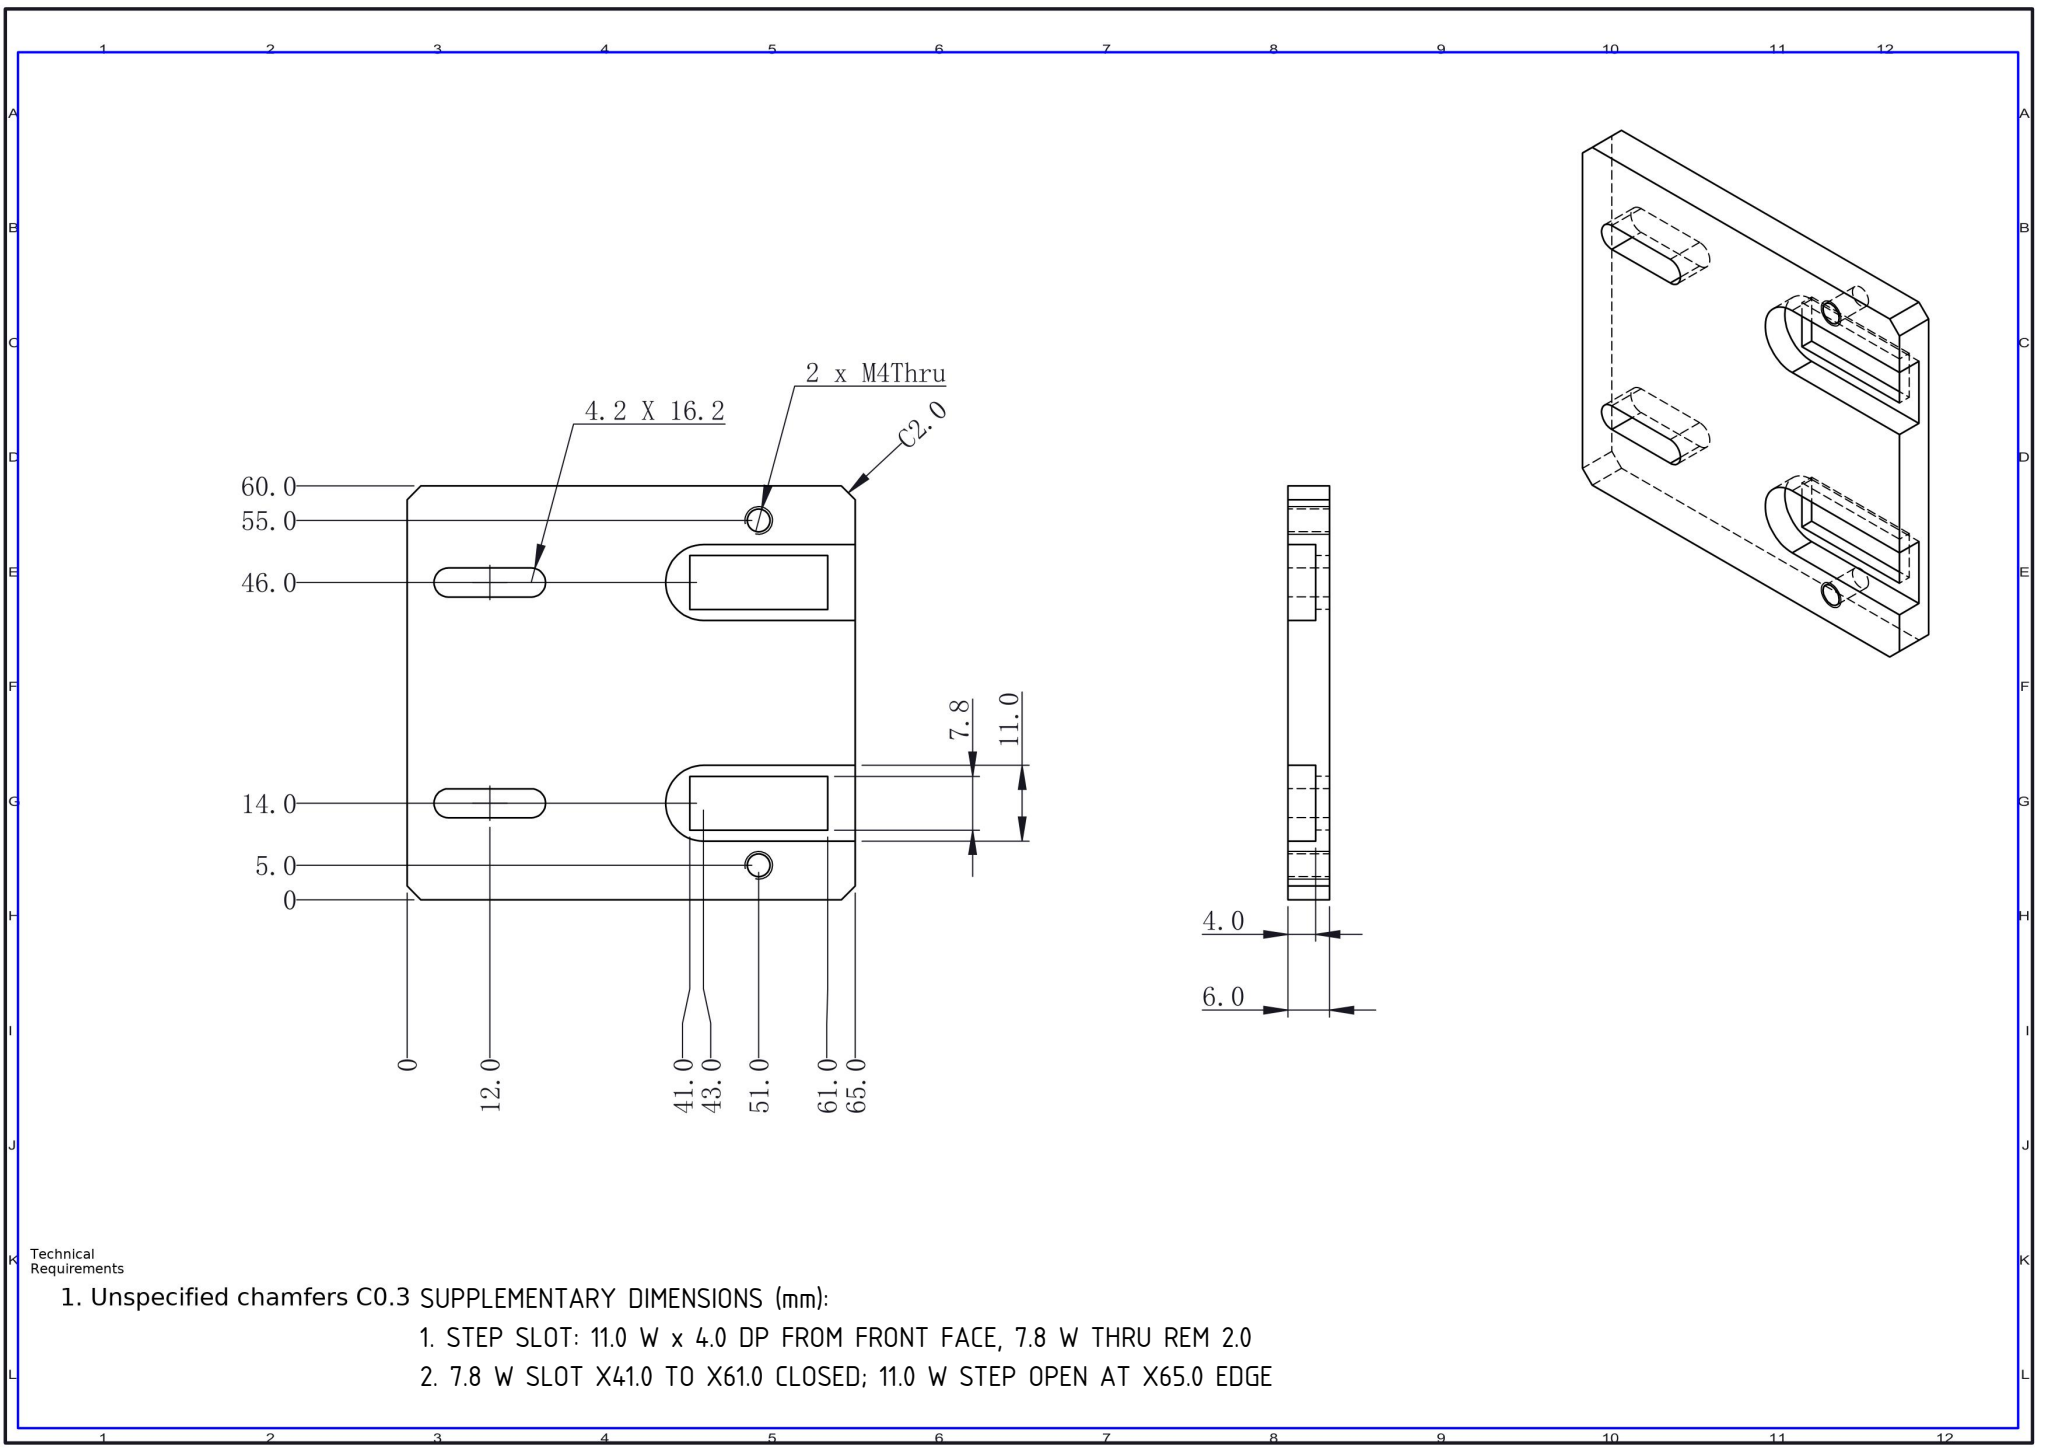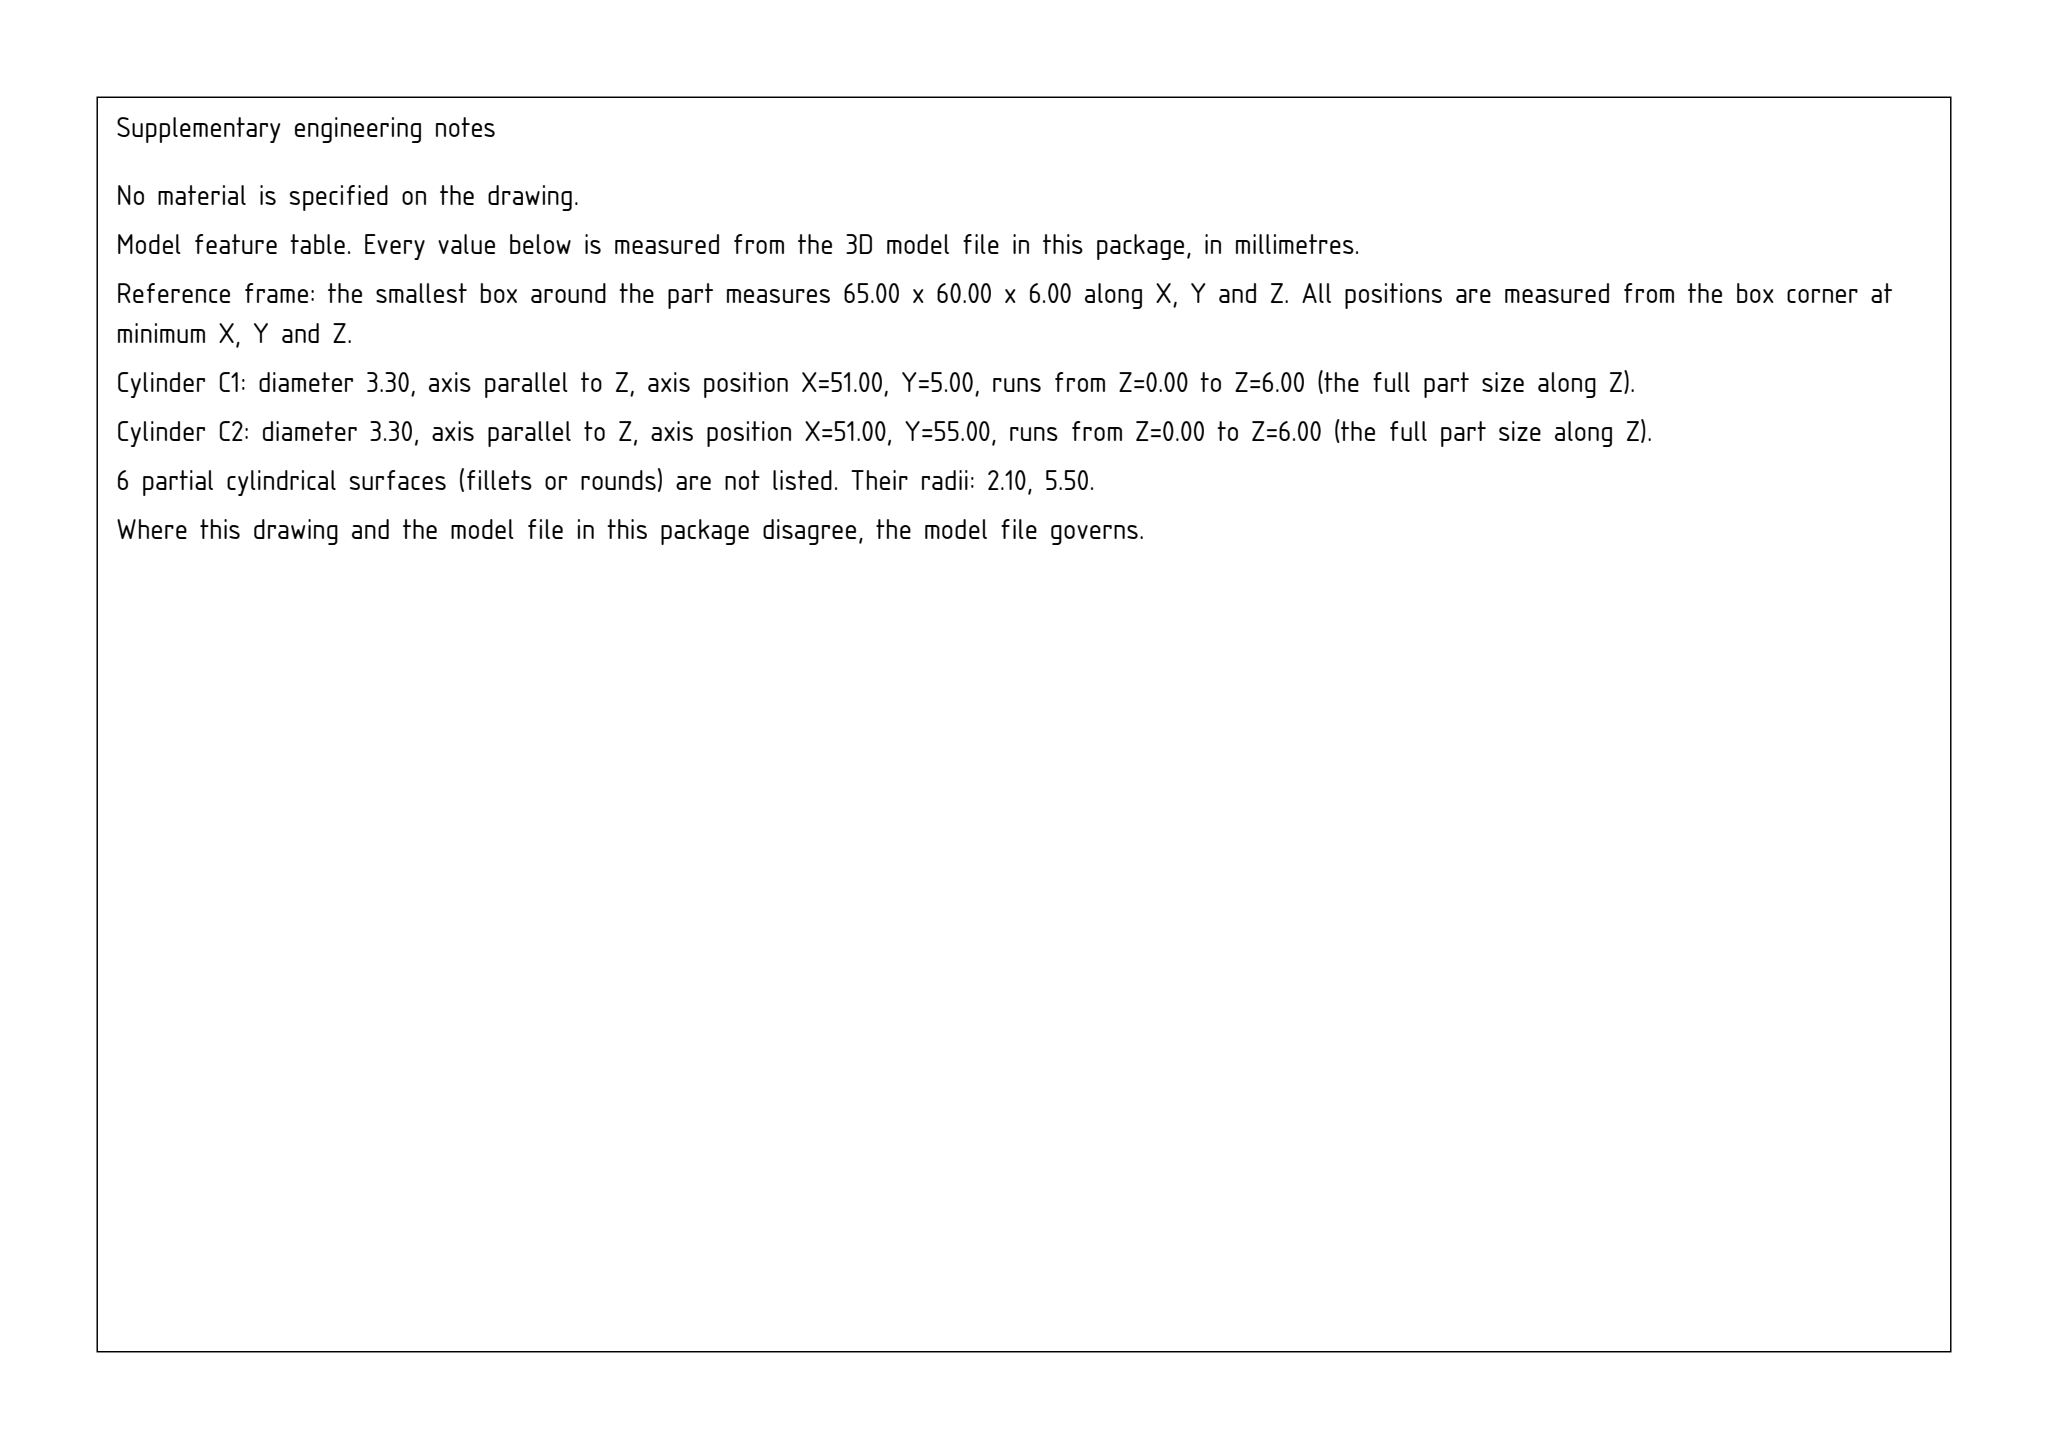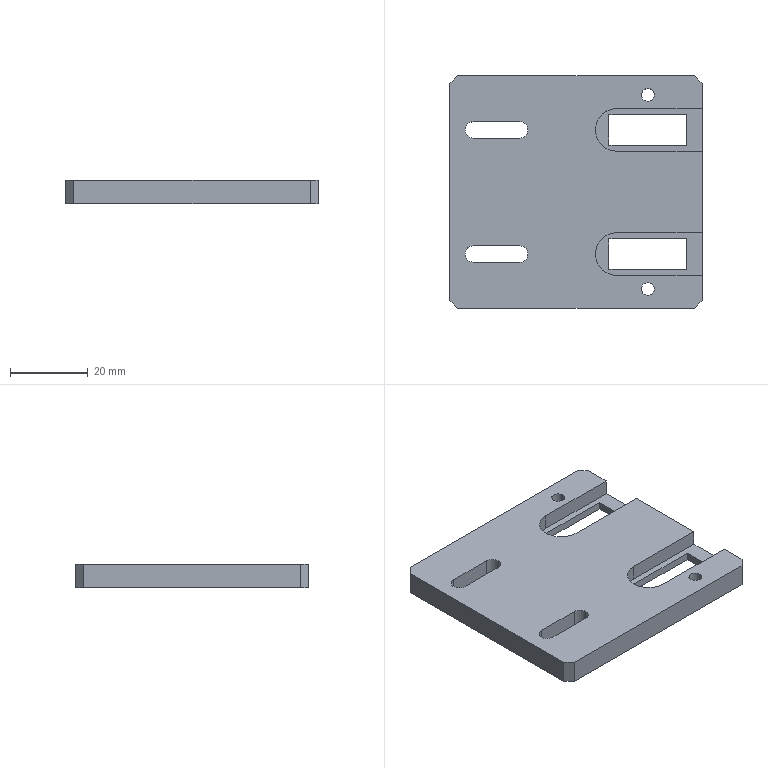Part | SolidWorks | mm | 1 solid | 40 faces | box 65 x 60 x 6 mm | volume 19538 mm3 | plane 28 | cylinder 12 | commonest cylinder face diameters 4.2 x6 3.3 x4 11 x2
build123d program:
from build123d import *

# Parameters (mm, degrees)
SKETCH1_W           = 65
SKETCH1_H           = 60
BOSS_EXTRUDE1_DEPTH = 6
CUT_EXTRUDE1_DEPTH  = 4
SKETCH3_W           = 20
SKETCH3_H           = 7.8
CUT_EXTRUDE2_DEPTH  = 89.549
CUT_EXTRUDE3_DEPTH  = 89.662
CHAMFER1_SIZE       = 2
M4_TAPPED_HOLE1_D   = 3.3


with BuildPart() as part:
    # Sketch1 → Boss-Extrude1 (new body)
    with BuildSketch(Plane.XY):
        with Locations((32.5, -30)):
            Rectangle(SKETCH1_W, SKETCH1_H)
    extrude(amount=BOSS_EXTRUDE1_DEPTH)

    # Sketch2 → Cut-Extrude1 (cut)
    with BuildSketch(Plane.XY.offset(6)):
        with BuildLine():
            Line((65, -19.5), (43, -19.5))
            ThreePointArc((43, -19.5), (37.5, -14), (43, -8.5))
            Line((43, -8.5), (65, -8.5))
            ThreePointArc((65, -8.5), (70.5, -14), (65, -19.5))
        make_face()
        with BuildLine():
            Line((65, -51.5), (43, -51.5))
            ThreePointArc((43, -51.5), (37.5, -46), (43, -40.5))
            Line((43, -40.5), (65, -40.5))
            ThreePointArc((65, -40.5), (70.5, -46), (65, -51.5))
        make_face()
    extrude(amount=-CUT_EXTRUDE1_DEPTH, mode=Mode.SUBTRACT)

    # Sketch3 → Cut-Extrude2 (cut, through all)
    with BuildSketch(Plane.XY.offset(2)):
        with Locations((51, -14)):
            Rectangle(SKETCH3_W, SKETCH3_H)
        with Locations((51, -46)):
            Rectangle(SKETCH3_W, SKETCH3_H)
    extrude(amount=-CUT_EXTRUDE2_DEPTH, mode=Mode.SUBTRACT)

    # Sketch4 → Cut-Extrude3 (cut, through all)
    with BuildSketch(Plane.XY.offset(6)):
        with BuildLine():
            Line((6, -11.9), (18, -11.9))
            ThreePointArc((18, -11.9), (20.1, -14), (18, -16.1))
            Line((18, -16.1), (6, -16.1))
            ThreePointArc((6, -16.1), (3.9, -14), (6, -11.9))
        make_face()
        with BuildLine():
            Line((6, -43.9), (18, -43.9))
            ThreePointArc((18, -43.9), (20.1, -46), (18, -48.1))
            Line((18, -48.1), (6, -48.1))
            ThreePointArc((6, -48.1), (3.9, -46), (6, -43.9))
        make_face()
    extrude(amount=-CUT_EXTRUDE3_DEPTH, mode=Mode.SUBTRACT)

    # Chamfer1
    chamfer1_edges = [part.edges().sort_by_distance(p)[0] for p in [
        (0, 0, 3),
        (65, 0, 3),
        (65, -60, 3),
        (0, -60, 3),
    ]]
    chamfer(chamfer1_edges, length=CHAMFER1_SIZE)

    # M4 Tapped Hole1 (through all)
    with Locations(Plane.XY.offset(6)):
        with Locations((51, -5), (51, -55)):
            Hole(M4_TAPPED_HOLE1_D / 2)


solid = part.part